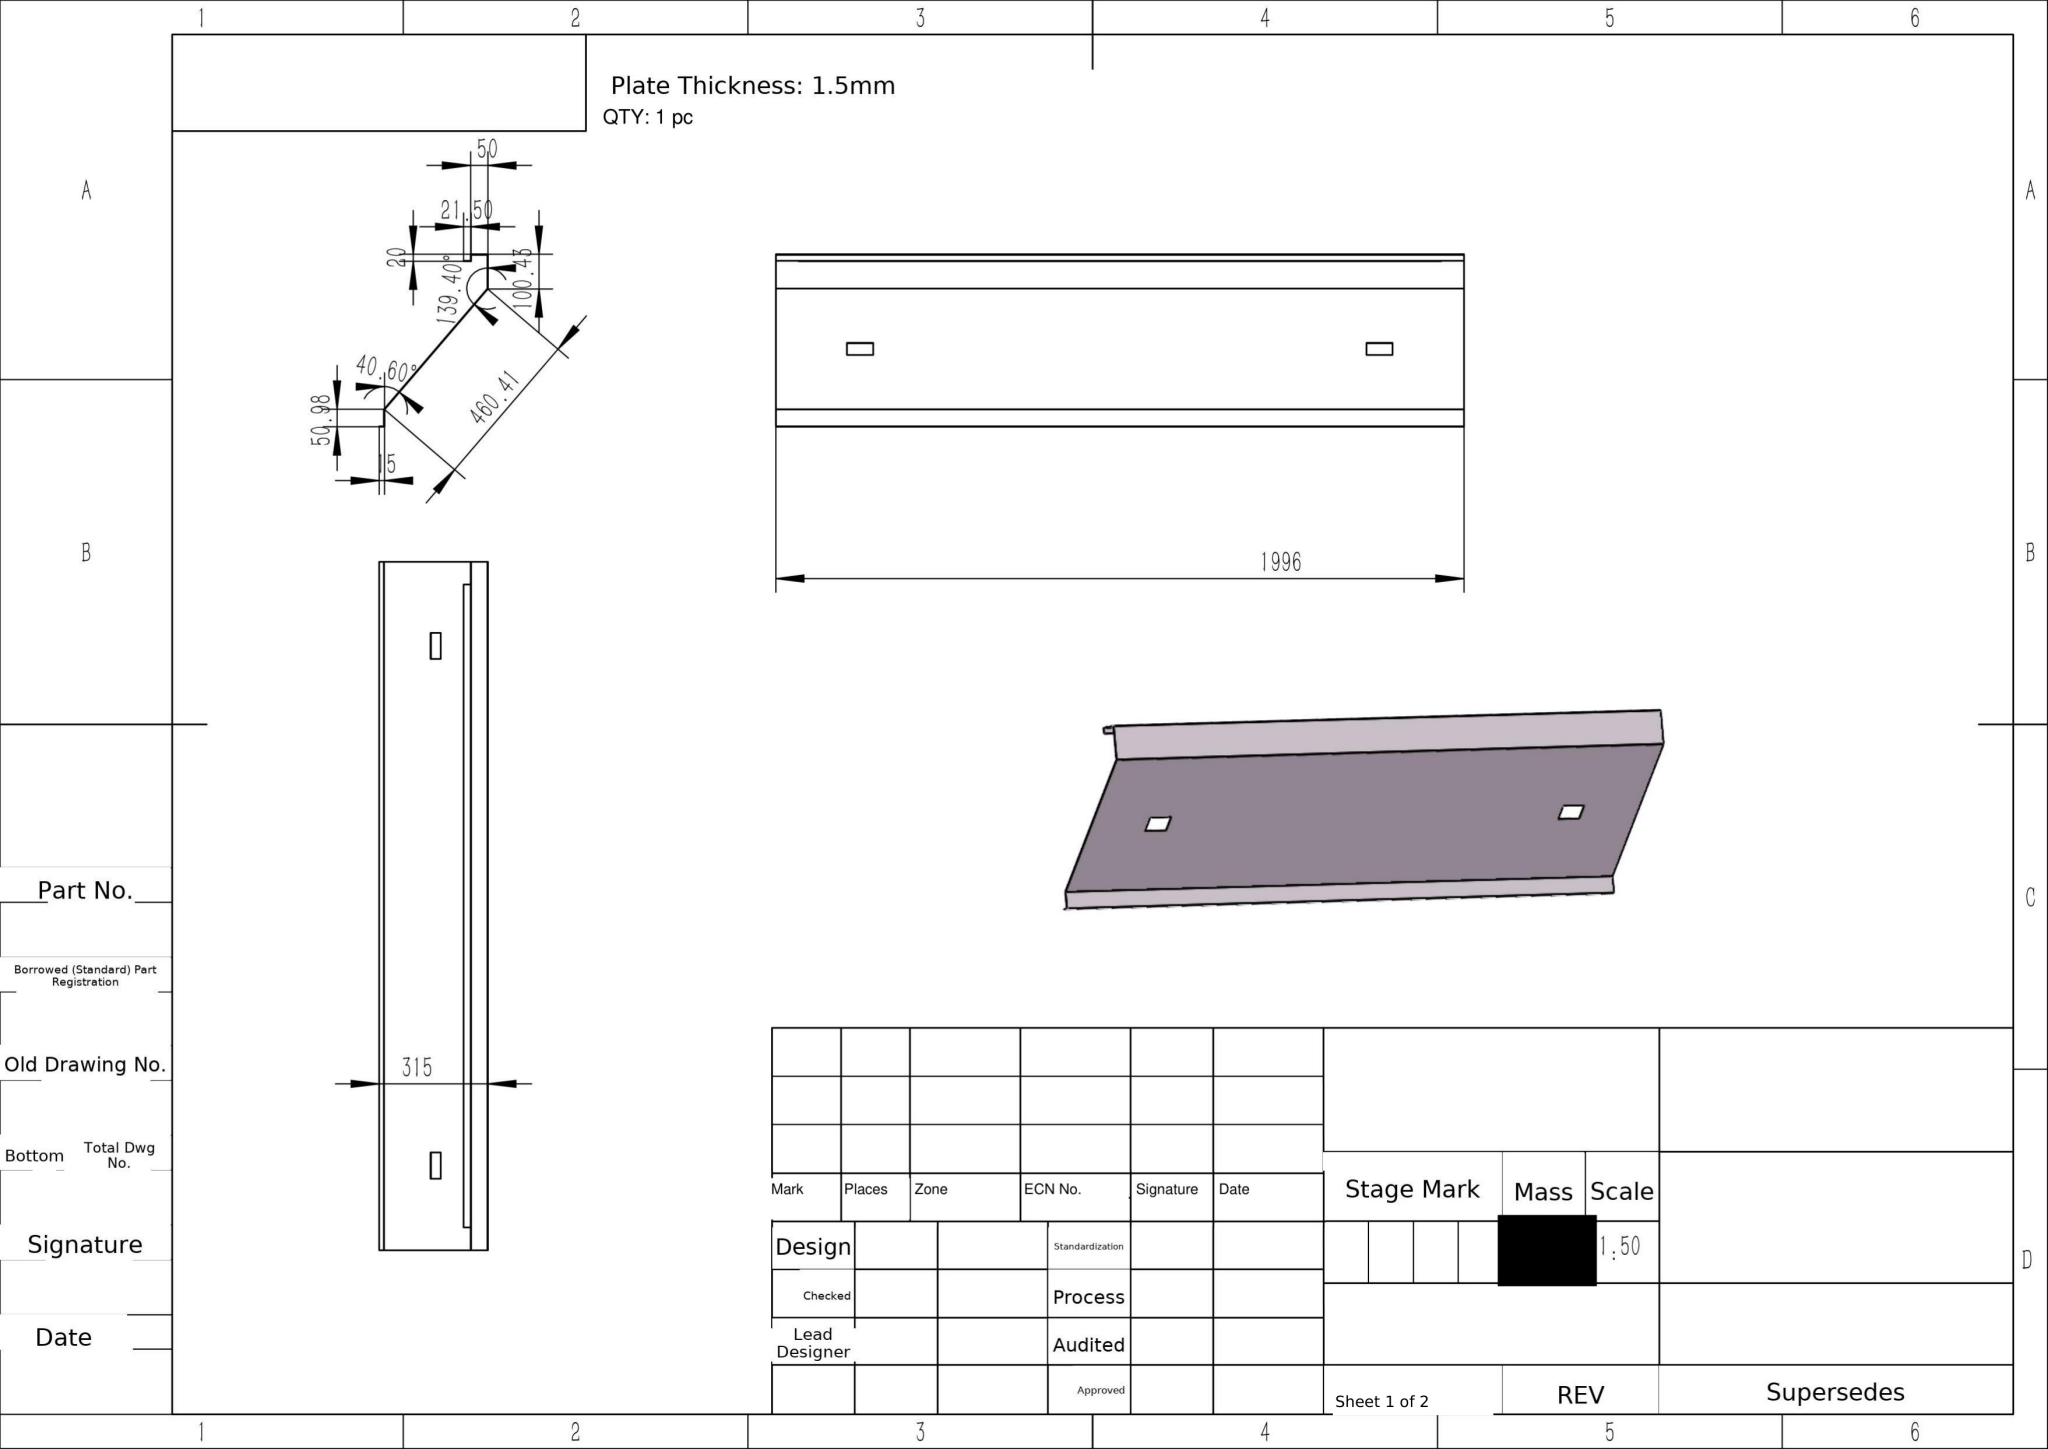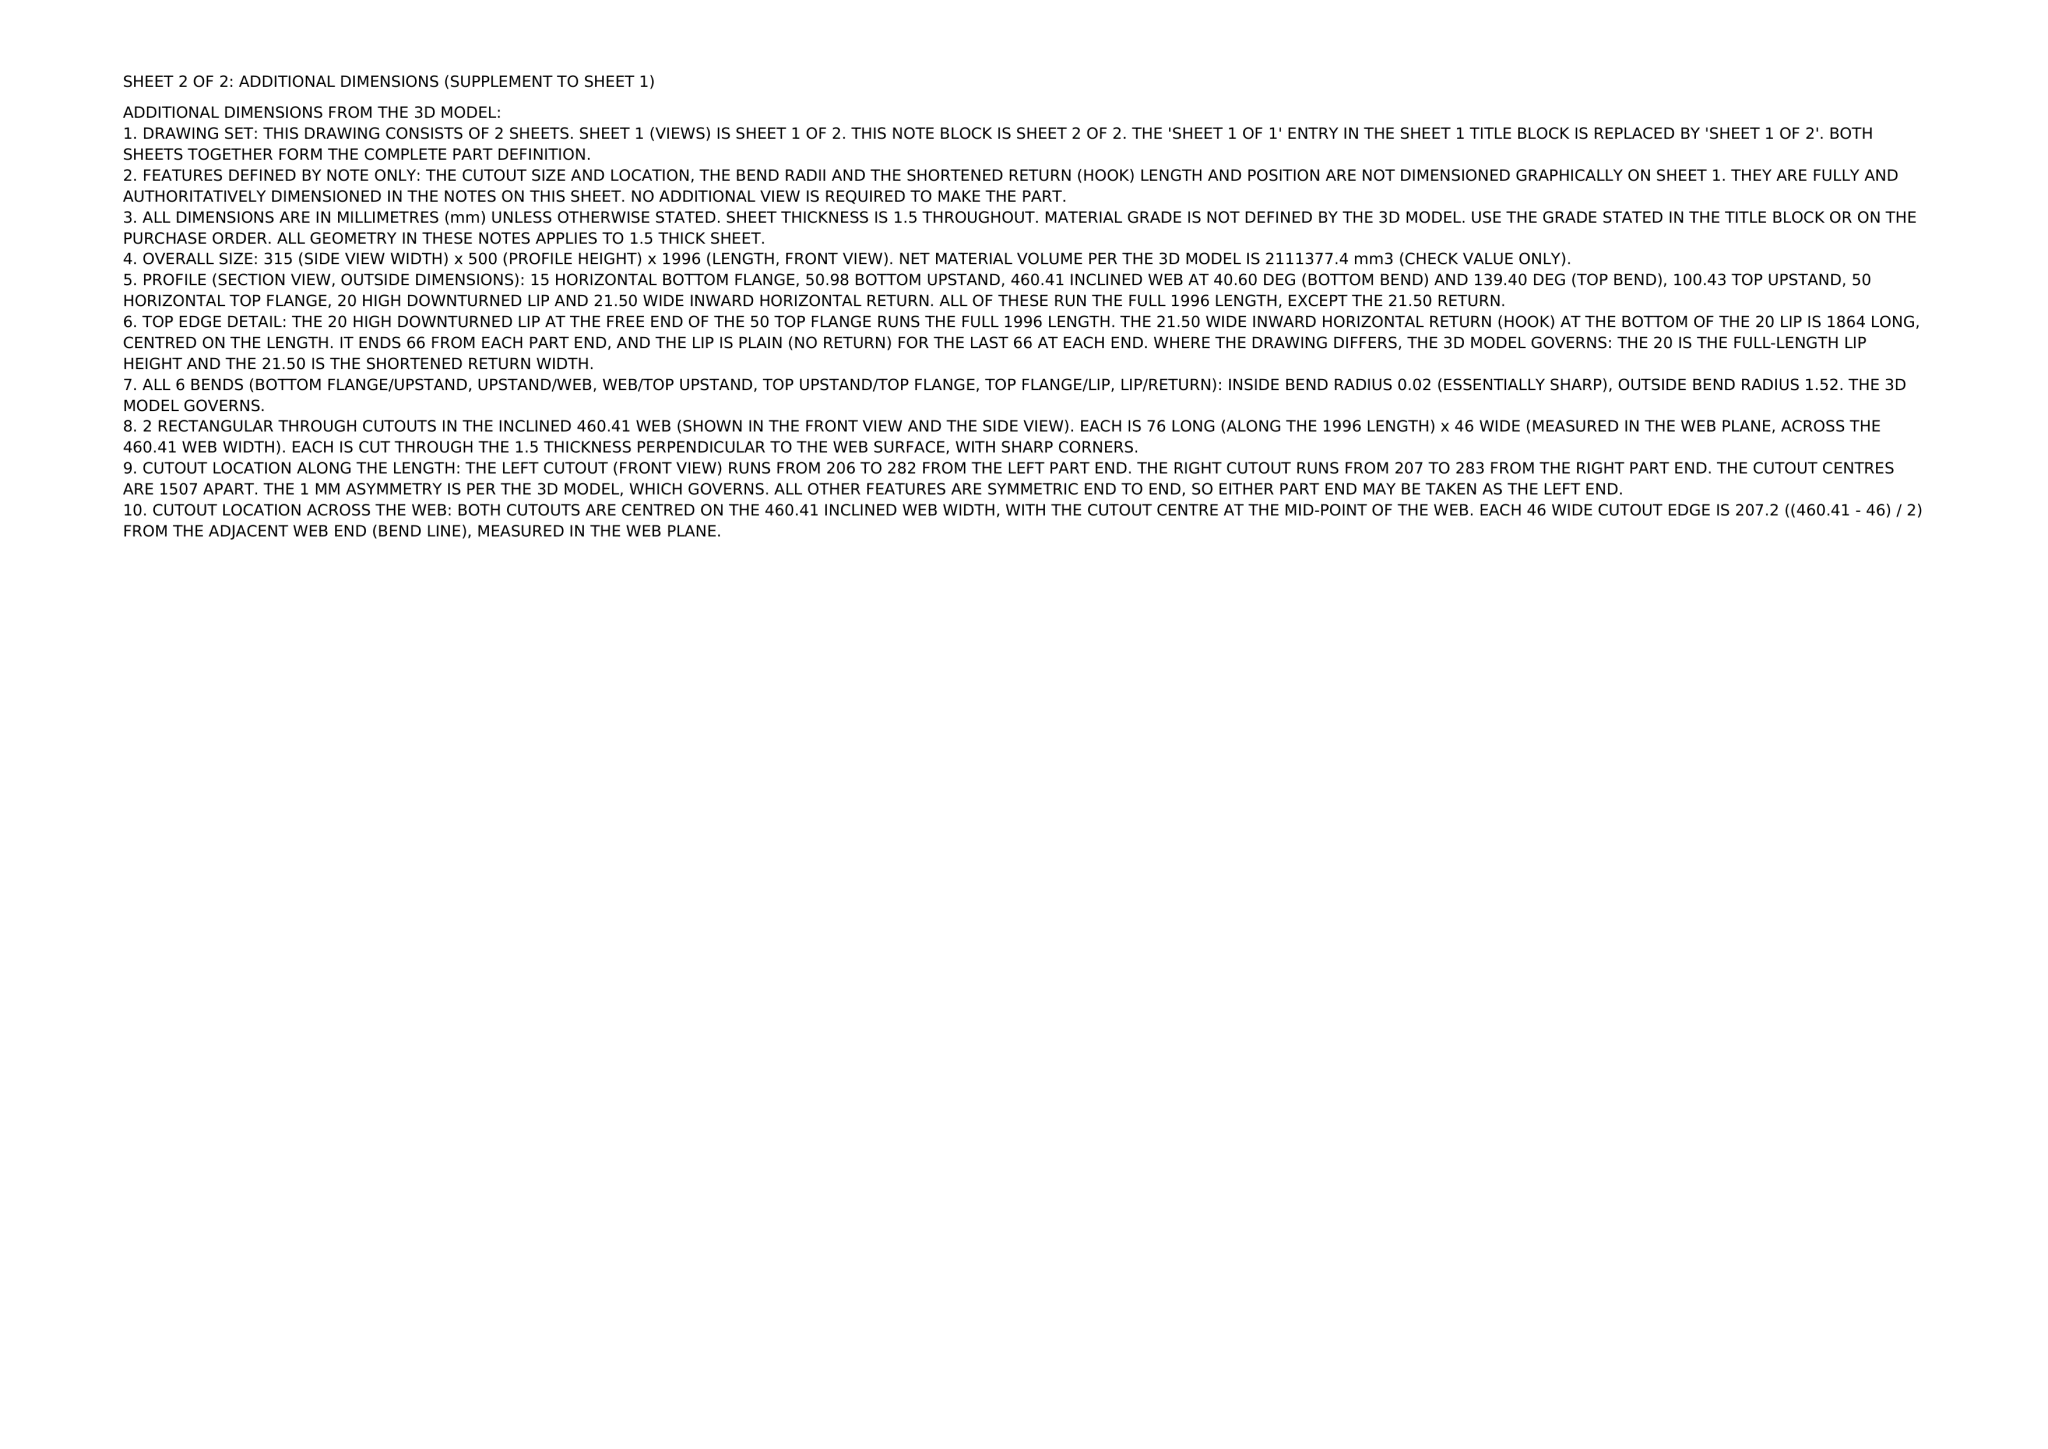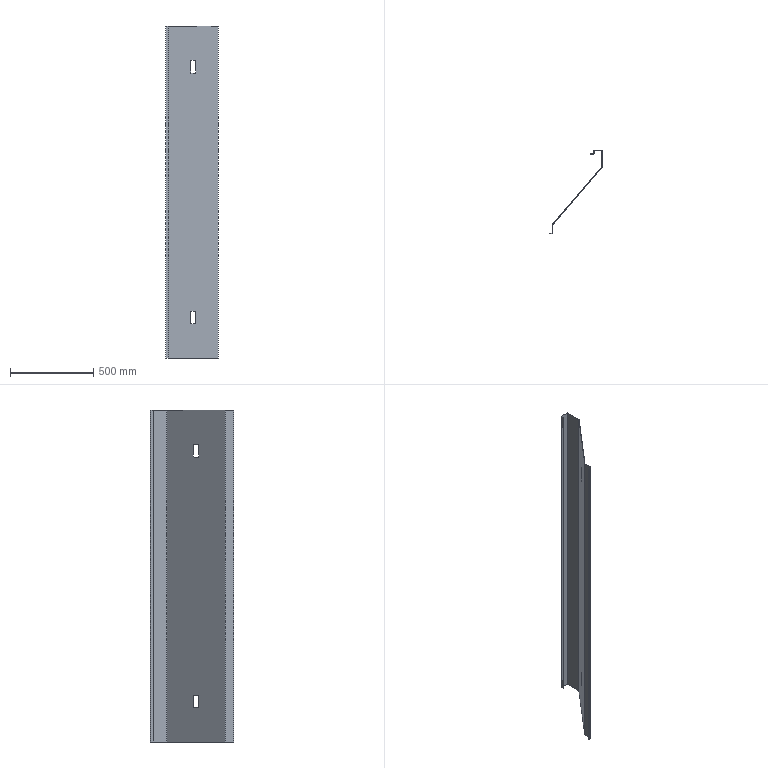Part | NX | mm | Notched Dual-Aperture Panel Plate | 1 solid | 52 faces | box 315 x 500 x 1996 mm | volume 2111377 mm3 | plane 40 | cylinder 12 | commonest cylinder face diameters 3.04 x6 0.04 x6